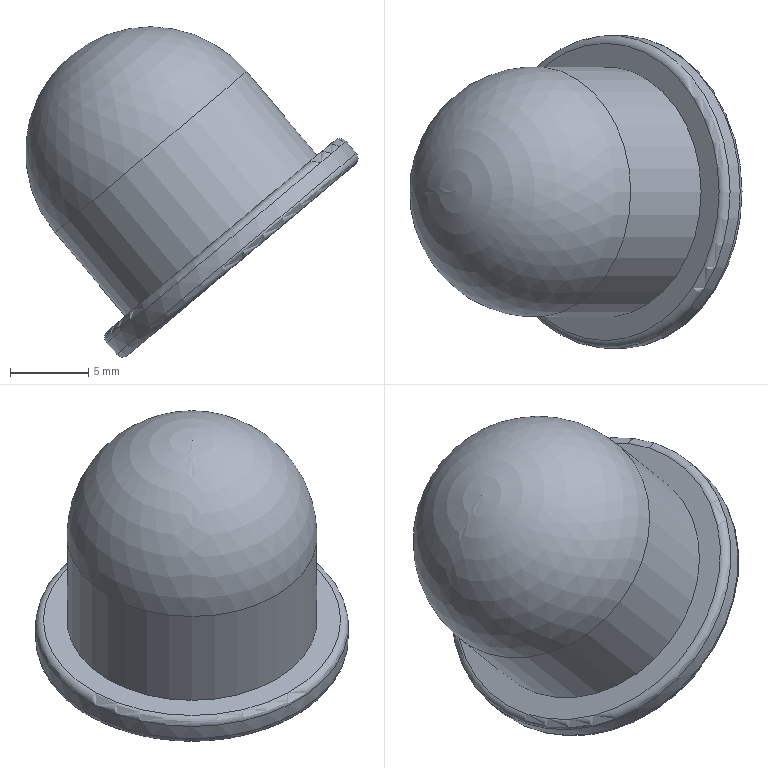Component | NX | PIVOTCUP | 1 solid | 10 faces | box 21.24 x 20 x 21.12 mm | volume 2204 mm3 | cylinder 3 | torus 3 | plane 2 | sphere 2 | commonest cylinder face diameters 16 x1 20 x1 10 x1
STEP:
#1=CARTESIAN_POINT('',(0.,0.,0.));
#2=DIRECTION('',(0.,0.,1.));
#3=DIRECTION('',(1.,0.,0.));
#4=AXIS2_PLACEMENT_3D('',#1,#2,#3);
#5=CARTESIAN_POINT('',(-459.062,-0.,-7.212));
#6=VERTEX_POINT('',#5);
#7=CARTESIAN_POINT('',(-471.318,-0.,-17.497));
#8=VERTEX_POINT('',#7);
#9=CARTESIAN_POINT('',(-465.19,-0.,-12.354));
#10=DIRECTION('',(0.6428,0.,-0.766));
#11=DIRECTION('',(0.766,0.,0.6428));
#12=AXIS2_PLACEMENT_3D('',#9,#10,#11);
#13=CIRCLE('',#12,8.);
#14=CARTESIAN_POINT('',(-470.332,-0.,-6.226));
#15=DIRECTION('',(0.6428,0.,-0.766));
#16=DIRECTION('',(0.766,0.,0.6428));
#17=AXIS2_PLACEMENT_3D('',#14,#15,#16);
#18=CYLINDRICAL_SURFACE('',#17,8.);
#19=CARTESIAN_POINT('',(0.,8.));
#20=DIRECTION('',(1.,0.));
#21=VECTOR('',#20,1.);
#22=LINE('',#19,#21);
#23=(GEOMETRIC_REPRESENTATION_CONTEXT(2)PARAMETRIC_REPRESENTATION_CONTEXT()REPRESENTATION_CONTEXT('',''));
#24=DEFINITIONAL_REPRESENTATION('',(#22),#23);
#25=PCURVE('',#18,#24);
#26=CARTESIAN_POINT('',(-465.19,-0.,-12.354));
#27=DIRECTION('',(-0.6428,0.,0.766));
#28=DIRECTION('',(-0.766,0.,-0.6428));
#29=AXIS2_PLACEMENT_3D('',#26,#27,#28);
#30=SPHERICAL_SURFACE('',#29,8.);
#31=CARTESIAN_POINT('',(3.142,-0.));
#32=CARTESIAN_POINT('',(3.046,0.));
#33=CARTESIAN_POINT('',(2.856,0.));
#34=CARTESIAN_POINT('',(2.57,-0.));
#35=CARTESIAN_POINT('',(2.285,-0.));
#36=CARTESIAN_POINT('',(1.999,-0.));
#37=CARTESIAN_POINT('',(1.714,-0.));
#38=CARTESIAN_POINT('',(1.428,0.));
#39=CARTESIAN_POINT('',(1.142,-0.));
#40=CARTESIAN_POINT('',(0.8568,0.));
#41=CARTESIAN_POINT('',(0.5712,0.));
#42=CARTESIAN_POINT('',(0.2856,-0.));
#43=CARTESIAN_POINT('',(0.,-0.));
#44=CARTESIAN_POINT('',(-0.2856,-0.));
#45=CARTESIAN_POINT('',(-0.5712,0.));
#46=CARTESIAN_POINT('',(-0.8568,0.));
#47=CARTESIAN_POINT('',(-1.142,-0.));
#48=CARTESIAN_POINT('',(-1.428,0.));
#49=CARTESIAN_POINT('',(-1.714,-0.));
#50=CARTESIAN_POINT('',(-1.999,-0.));
#51=CARTESIAN_POINT('',(-2.285,-0.));
#52=CARTESIAN_POINT('',(-2.57,-0.));
#53=CARTESIAN_POINT('',(-2.856,0.));
#54=CARTESIAN_POINT('',(-3.046,0.));
#55=CARTESIAN_POINT('',(-3.142,-0.));
#56=B_SPLINE_CURVE_WITH_KNOTS('',3,(#31,#32,#33,#34,#35,#36,#37,#38,#39,#40,#41,#42,#43,#44,#45,#46,#47,#48,#49,#50,#51,#52,#53,#54,#55),.UNSPECIFIED.,.F.,.F.,(4,1,1,1,1,1,1,1,1,1,1,1,1,1,1,1,1,1,1,1,1,1,4),(0.,0.2856,0.5712,0.8568,1.142,1.428,1.714,1.999,2.285,2.57,2.856,3.142,3.427,3.713,3.998,4.284,4.57,4.855,5.141,5.426,5.712,5.998,6.283),.QUASI_UNIFORM_KNOTS.);
#57=(GEOMETRIC_REPRESENTATION_CONTEXT(2)PARAMETRIC_REPRESENTATION_CONTEXT()REPRESENTATION_CONTEXT('',''));
#58=DEFINITIONAL_REPRESENTATION('',(#56),#57);
#59=PCURVE('',#30,#58);
#60=SURFACE_CURVE('',#13,(#25,#59),.PCURVE_S1.);
#61=EDGE_CURVE('',#6,#8,#60,.T.);
#62=ORIENTED_EDGE('',*,*,#61,.T.);
#63=CARTESIAN_POINT('',(-465.19,-0.,-12.354));
#64=DIRECTION('',(0.6428,0.,-0.766));
#65=DIRECTION('',(0.766,0.,0.6428));
#66=AXIS2_PLACEMENT_3D('',#63,#64,#65);
#67=CIRCLE('',#66,8.);
#68=CARTESIAN_POINT('',(0.,8.));
#69=DIRECTION('',(1.,0.));
#70=VECTOR('',#69,1.);
#71=LINE('',#68,#70);
#72=(GEOMETRIC_REPRESENTATION_CONTEXT(2)PARAMETRIC_REPRESENTATION_CONTEXT()REPRESENTATION_CONTEXT('',''));
#73=DEFINITIONAL_REPRESENTATION('',(#71),#72);
#74=PCURVE('',#18,#73);
#75=CARTESIAN_POINT('',(9.425,-0.));
#76=CARTESIAN_POINT('',(9.33,0.));
#77=CARTESIAN_POINT('',(9.139,0.));
#78=CARTESIAN_POINT('',(8.854,-0.));
#79=CARTESIAN_POINT('',(8.568,-0.));
#80=CARTESIAN_POINT('',(8.282,-0.));
#81=CARTESIAN_POINT('',(7.997,-0.));
#82=CARTESIAN_POINT('',(7.711,0.));
#83=CARTESIAN_POINT('',(7.426,-0.));
#84=CARTESIAN_POINT('',(7.14,0.));
#85=CARTESIAN_POINT('',(6.854,0.));
#86=CARTESIAN_POINT('',(6.569,-0.));
#87=CARTESIAN_POINT('',(6.283,-0.));
#88=CARTESIAN_POINT('',(5.998,-0.));
#89=CARTESIAN_POINT('',(5.712,0.));
#90=CARTESIAN_POINT('',(5.426,0.));
#91=CARTESIAN_POINT('',(5.141,-0.));
#92=CARTESIAN_POINT('',(4.855,0.));
#93=CARTESIAN_POINT('',(4.57,-0.));
#94=CARTESIAN_POINT('',(4.284,-0.));
#95=CARTESIAN_POINT('',(3.998,-0.));
#96=CARTESIAN_POINT('',(3.713,-0.));
#97=CARTESIAN_POINT('',(3.427,0.));
#98=CARTESIAN_POINT('',(3.237,0.));
#99=CARTESIAN_POINT('',(3.142,-0.));
#100=B_SPLINE_CURVE_WITH_KNOTS('',3,(#75,#76,#77,#78,#79,#80,#81,#82,#83,#84,#85,#86,#87,#88,#89,#90,#91,#92,#93,#94,#95,#96,#97,#98,#99),.UNSPECIFIED.,.F.,.F.,(4,1,1,1,1,1,1,1,1,1,1,1,1,1,1,1,1,1,1,1,1,1,4),(0.,0.2856,0.5712,0.8568,1.142,1.428,1.714,1.999,2.285,2.57,2.856,3.142,3.427,3.713,3.998,4.284,4.57,4.855,5.141,5.426,5.712,5.998,6.283),.QUASI_UNIFORM_KNOTS.);
#101=(GEOMETRIC_REPRESENTATION_CONTEXT(2)PARAMETRIC_REPRESENTATION_CONTEXT()REPRESENTATION_CONTEXT('',''));
#102=DEFINITIONAL_REPRESENTATION('',(#100),#101);
#103=PCURVE('',#30,#102);
#104=SURFACE_CURVE('',#67,(#74,#103),.PCURVE_S1.);
#105=EDGE_CURVE('',#8,#6,#104,.T.);
#106=ORIENTED_EDGE('',*,*,#105,.T.);
#107=CARTESIAN_POINT('',(-454.562,-0.,-12.574));
#108=VERTEX_POINT('',#107);
#109=CARTESIAN_POINT('',(-459.062,-0.,-7.212));
#110=CARTESIAN_POINT('',(-454.562,-0.,-12.574));
#111=B_SPLINE_CURVE_WITH_KNOTS('',1,(#109,#110),.UNSPECIFIED.,.F.,.F.,(2,2),(8.,15.),.PIECEWISE_BEZIER_KNOTS.);
#112=CARTESIAN_POINT('',(6.283,0.));
#113=DIRECTION('',(0.,1.));
#114=VECTOR('',#113,1.);
#115=LINE('',#112,#114);
#116=(GEOMETRIC_REPRESENTATION_CONTEXT(2)PARAMETRIC_REPRESENTATION_CONTEXT()REPRESENTATION_CONTEXT('',''));
#117=DEFINITIONAL_REPRESENTATION('',(#115),#116);
#118=PCURVE('',#18,#117);
#119=CARTESIAN_POINT('',(0.,0.));
#120=DIRECTION('',(0.,1.));
#121=VECTOR('',#120,1.);
#122=LINE('',#119,#121);
#123=(GEOMETRIC_REPRESENTATION_CONTEXT(2)PARAMETRIC_REPRESENTATION_CONTEXT()REPRESENTATION_CONTEXT('',''));
#124=DEFINITIONAL_REPRESENTATION('',(#122),#123);
#125=PCURVE('',#18,#124);
#126=SEAM_CURVE('',#111,(#118,#125),.PCURVE_S1.);
#127=EDGE_CURVE('',#6,#108,#126,.T.);
#128=ORIENTED_EDGE('',*,*,#127,.T.);
#129=CARTESIAN_POINT('',(-466.819,-0.,-22.859));
#130=VERTEX_POINT('',#129);
#131=CARTESIAN_POINT('',(-460.69,-0.,-17.717));
#132=DIRECTION('',(0.6428,0.,-0.766));
#133=DIRECTION('',(-0.766,0.,-0.6428));
#134=AXIS2_PLACEMENT_3D('',#131,#132,#133);
#135=CIRCLE('',#134,8.);
#136=CARTESIAN_POINT('',(3.142,15.));
#137=DIRECTION('',(1.,0.));
#138=VECTOR('',#137,1.);
#139=LINE('',#136,#138);
#140=(GEOMETRIC_REPRESENTATION_CONTEXT(2)PARAMETRIC_REPRESENTATION_CONTEXT()REPRESENTATION_CONTEXT('',''));
#141=DEFINITIONAL_REPRESENTATION('',(#139),#140);
#142=PCURVE('',#18,#141);
#143=CARTESIAN_POINT('',(-460.69,-0.,-17.717));
#144=DIRECTION('',(-0.6428,0.,0.766));
#145=DIRECTION('',(-0.766,0.,-0.6428));
#146=AXIS2_PLACEMENT_3D('',#143,#144,#145);
#147=PLANE('',#146);
#148=CARTESIAN_POINT('',(8.,0.));
#149=CARTESIAN_POINT('',(8.,-13.856));
#150=CARTESIAN_POINT('',(-4.,-6.928));
#151=CARTESIAN_POINT('',(-16.,-0.));
#152=CARTESIAN_POINT('',(-4.,6.928));
#153=CARTESIAN_POINT('',(8.,13.856));
#154=CARTESIAN_POINT('',(8.,0.));
#155=(BOUNDED_CURVE()B_SPLINE_CURVE(2,(#148,#149,#150,#151,#152,#153,#154),.UNSPECIFIED.,.T.,.F.)B_SPLINE_CURVE_WITH_KNOTS((1,2,2,2,2,1),(-2.094,0.,2.094,4.189,6.283,8.378),.UNSPECIFIED.)CURVE()GEOMETRIC_REPRESENTATION_ITEM()RATIONAL_B_SPLINE_CURVE((1.,0.5,1.,0.5,1.,0.5,1.))REPRESENTATION_ITEM(''));
#156=(GEOMETRIC_REPRESENTATION_CONTEXT(2)PARAMETRIC_REPRESENTATION_CONTEXT()REPRESENTATION_CONTEXT('',''));
#157=DEFINITIONAL_REPRESENTATION('',(#155),#156);
#158=PCURVE('',#147,#157);
#159=SURFACE_CURVE('',#135,(#142,#158),.PCURVE_S1.);
#160=EDGE_CURVE('',#130,#108,#159,.T.);
#161=ORIENTED_EDGE('',*,*,#160,.F.);
#162=CARTESIAN_POINT('',(-460.69,-0.,-17.717));
#163=DIRECTION('',(0.6428,0.,-0.766));
#164=DIRECTION('',(-0.766,0.,-0.6428));
#165=AXIS2_PLACEMENT_3D('',#162,#163,#164);
#166=CIRCLE('',#165,8.);
#167=CARTESIAN_POINT('',(-3.142,15.));
#168=DIRECTION('',(1.,0.));
#169=VECTOR('',#168,1.);
#170=LINE('',#167,#169);
#171=(GEOMETRIC_REPRESENTATION_CONTEXT(2)PARAMETRIC_REPRESENTATION_CONTEXT()REPRESENTATION_CONTEXT('',''));
#172=DEFINITIONAL_REPRESENTATION('',(#170),#171);
#173=PCURVE('',#18,#172);
#174=CARTESIAN_POINT('',(8.,0.));
#175=CARTESIAN_POINT('',(8.,-13.856));
#176=CARTESIAN_POINT('',(-4.,-6.928));
#177=CARTESIAN_POINT('',(-16.,-0.));
#178=CARTESIAN_POINT('',(-4.,6.928));
#179=CARTESIAN_POINT('',(8.,13.856));
#180=CARTESIAN_POINT('',(8.,0.));
#181=(BOUNDED_CURVE()B_SPLINE_CURVE(2,(#174,#175,#176,#177,#178,#179,#180),.UNSPECIFIED.,.T.,.F.)B_SPLINE_CURVE_WITH_KNOTS((1,2,2,2,2,1),(-2.094,0.,2.094,4.189,6.283,8.378),.UNSPECIFIED.)CURVE()GEOMETRIC_REPRESENTATION_ITEM()RATIONAL_B_SPLINE_CURVE((1.,0.5,1.,0.5,1.,0.5,1.))REPRESENTATION_ITEM(''));
#182=(GEOMETRIC_REPRESENTATION_CONTEXT(2)PARAMETRIC_REPRESENTATION_CONTEXT()REPRESENTATION_CONTEXT('',''));
#183=DEFINITIONAL_REPRESENTATION('',(#181),#182);
#184=PCURVE('',#147,#183);
#185=SURFACE_CURVE('',#166,(#173,#184),.PCURVE_S1.);
#186=EDGE_CURVE('',#108,#130,#185,.T.);
#187=ORIENTED_EDGE('',*,*,#186,.F.);
#188=ORIENTED_EDGE('',*,*,#127,.F.);
#189=EDGE_LOOP('',(#62,#106,#128,#161,#187,#188));
#190=FACE_BOUND('',#189,.T.);
#191=ADVANCED_FACE('',(#190),#18,.T.);
#192=CARTESIAN_POINT('',(-454.809,-0.,-15.392));
#193=VERTEX_POINT('',#192);
#194=CARTESIAN_POINT('',(-459.405,-0.,-19.249));
#195=DIRECTION('',(-0.6428,0.,0.766));
#196=DIRECTION('',(0.766,0.,0.6428));
#197=AXIS2_PLACEMENT_3D('',#194,#195,#196);
#198=CIRCLE('',#197,6.);
#199=CARTESIAN_POINT('',(-459.405,-0.,-19.249));
#200=DIRECTION('',(0.6428,0.,-0.766));
#201=DIRECTION('',(0.766,0.,0.6428));
#202=AXIS2_PLACEMENT_3D('',#199,#200,#201);
#203=PLANE('',#202);
#204=CARTESIAN_POINT('',(6.,0.));
#205=CARTESIAN_POINT('',(6.,-10.392));
#206=CARTESIAN_POINT('',(-3.,-5.196));
#207=CARTESIAN_POINT('',(-12.,-0.));
#208=CARTESIAN_POINT('',(-3.,5.196));
#209=CARTESIAN_POINT('',(6.,10.392));
#210=CARTESIAN_POINT('',(6.,0.));
#211=(BOUNDED_CURVE()B_SPLINE_CURVE(2,(#204,#205,#206,#207,#208,#209,#210),.UNSPECIFIED.,.T.,.F.)B_SPLINE_CURVE_WITH_KNOTS((1,2,2,2,2,1),(-2.094,0.,2.094,4.189,6.283,8.378),.UNSPECIFIED.)CURVE()GEOMETRIC_REPRESENTATION_ITEM()RATIONAL_B_SPLINE_CURVE((1.,0.5,1.,0.5,1.,0.5,1.))REPRESENTATION_ITEM(''));
#212=(GEOMETRIC_REPRESENTATION_CONTEXT(2)PARAMETRIC_REPRESENTATION_CONTEXT()REPRESENTATION_CONTEXT('',''));
#213=DEFINITIONAL_REPRESENTATION('',(#211),#212);
#214=PCURVE('',#203,#213);
#215=CARTESIAN_POINT('',(-460.048,-0.,-18.483));
#216=DIRECTION('',(0.6428,0.,-0.766));
#217=DIRECTION('',(0.766,0.,0.6428));
#218=AXIS2_PLACEMENT_3D('',#215,#216,#217);
#219=TOROIDAL_SURFACE('',#218,6.,1.);
#220=CARTESIAN_POINT('',(6.283,7.854));
#221=DIRECTION('',(-1.,0.));
#222=VECTOR('',#221,1.);
#223=LINE('',#220,#222);
#224=(GEOMETRIC_REPRESENTATION_CONTEXT(2)PARAMETRIC_REPRESENTATION_CONTEXT()REPRESENTATION_CONTEXT('',''));
#225=DEFINITIONAL_REPRESENTATION('',(#223),#224);
#226=PCURVE('',#219,#225);
#227=SURFACE_CURVE('',#198,(#214,#226),.PCURVE_S1.);
#228=EDGE_CURVE('',#193,#193,#227,.T.);
#229=ORIENTED_EDGE('',*,*,#228,.T.);
#230=EDGE_LOOP('',(#229));
#231=FACE_BOUND('',#230,.T.);
#232=CARTESIAN_POINT('',(-452.127,-0.,-13.142));
#233=VERTEX_POINT('',#232);
#234=CARTESIAN_POINT('',(-459.405,-0.,-19.249));
#235=DIRECTION('',(0.6428,0.,-0.766));
#236=DIRECTION('',(0.766,0.,0.6428));
#237=AXIS2_PLACEMENT_3D('',#234,#235,#236);
#238=CIRCLE('',#237,9.5);
#239=CARTESIAN_POINT('',(0.,0.));
#240=DIRECTION('',(1.,0.));
#241=AXIS2_PLACEMENT_2D('',#239,#240);
#242=CIRCLE('',#241,9.5);
#243=(GEOMETRIC_REPRESENTATION_CONTEXT(2)PARAMETRIC_REPRESENTATION_CONTEXT()REPRESENTATION_CONTEXT('',''));
#244=DEFINITIONAL_REPRESENTATION('',(#242),#243);
#245=PCURVE('',#203,#244);
#246=CARTESIAN_POINT('',(-459.726,-0.,-18.866));
#247=DIRECTION('',(0.6428,0.,-0.766));
#248=DIRECTION('',(0.766,0.,0.6428));
#249=AXIS2_PLACEMENT_3D('',#246,#247,#248);
#250=TOROIDAL_SURFACE('',#249,9.5,0.5);
#251=CARTESIAN_POINT('',(0.,7.854));
#252=DIRECTION('',(1.,0.));
#253=VECTOR('',#252,1.);
#254=LINE('',#251,#253);
#255=(GEOMETRIC_REPRESENTATION_CONTEXT(2)PARAMETRIC_REPRESENTATION_CONTEXT()REPRESENTATION_CONTEXT('',''));
#256=DEFINITIONAL_REPRESENTATION('',(#254),#255);
#257=PCURVE('',#250,#256);
#258=SURFACE_CURVE('',#238,(#245,#257),.PCURVE_S1.);
#259=EDGE_CURVE('',#233,#233,#258,.T.);
#260=ORIENTED_EDGE('',*,*,#259,.T.);
#261=EDGE_LOOP('',(#260));
#262=FACE_BOUND('',#261,.T.);
#263=ADVANCED_FACE('',(#231,#262),#203,.T.);
#264=CARTESIAN_POINT('',(-467.968,-0.,-23.823));
#265=VERTEX_POINT('',#264);
#266=CARTESIAN_POINT('',(-460.69,-0.,-17.717));
#267=DIRECTION('',(-0.6428,0.,0.766));
#268=DIRECTION('',(-0.766,0.,-0.6428));
#269=AXIS2_PLACEMENT_3D('',#266,#267,#268);
#270=CIRCLE('',#269,9.5);
#271=CARTESIAN_POINT('',(0.,0.));
#272=DIRECTION('',(1.,0.));
#273=AXIS2_PLACEMENT_2D('',#271,#272);
#274=CIRCLE('',#273,9.5);
#275=(GEOMETRIC_REPRESENTATION_CONTEXT(2)PARAMETRIC_REPRESENTATION_CONTEXT()REPRESENTATION_CONTEXT('',''));
#276=DEFINITIONAL_REPRESENTATION('',(#274),#275);
#277=PCURVE('',#147,#276);
#278=CARTESIAN_POINT('',(-460.369,-0.,-18.1));
#279=DIRECTION('',(-0.6428,0.,0.766));
#280=DIRECTION('',(-0.766,0.,-0.6428));
#281=AXIS2_PLACEMENT_3D('',#278,#279,#280);
#282=TOROIDAL_SURFACE('',#281,9.5,0.5);
#283=CARTESIAN_POINT('',(0.,7.854));
#284=DIRECTION('',(1.,0.));
#285=VECTOR('',#284,1.);
#286=LINE('',#283,#285);
#287=(GEOMETRIC_REPRESENTATION_CONTEXT(2)PARAMETRIC_REPRESENTATION_CONTEXT()REPRESENTATION_CONTEXT('',''));
#288=DEFINITIONAL_REPRESENTATION('',(#286),#287);
#289=PCURVE('',#282,#288);
#290=SURFACE_CURVE('',#270,(#277,#289),.PCURVE_S1.);
#291=EDGE_CURVE('',#265,#265,#290,.T.);
#292=ORIENTED_EDGE('',*,*,#291,.T.);
#293=EDGE_LOOP('',(#292));
#294=FACE_BOUND('',#293,.T.);
#295=ORIENTED_EDGE('',*,*,#160,.T.);
#296=ORIENTED_EDGE('',*,*,#186,.T.);
#297=EDGE_LOOP('',(#295,#296));
#298=FACE_BOUND('',#297,.T.);
#299=ADVANCED_FACE('',(#294,#298),#147,.T.);
#300=CARTESIAN_POINT('',(-452.066,-0.,-12.438));
#301=VERTEX_POINT('',#300);
#302=CARTESIAN_POINT('',(-459.726,-0.,-18.866));
#303=DIRECTION('',(-0.6428,0.,0.766));
#304=DIRECTION('',(0.766,0.,0.6428));
#305=AXIS2_PLACEMENT_3D('',#302,#303,#304);
#306=CIRCLE('',#305,10.);
#307=CARTESIAN_POINT('',(-460.69,-0.,-17.717));
#308=DIRECTION('',(0.6428,0.,-0.766));
#309=DIRECTION('',(0.766,0.,0.6428));
#310=AXIS2_PLACEMENT_3D('',#307,#308,#309);
#311=CYLINDRICAL_SURFACE('',#310,10.);
#312=CARTESIAN_POINT('',(6.283,1.5));
#313=DIRECTION('',(-1.,0.));
#314=VECTOR('',#313,1.);
#315=LINE('',#312,#314);
#316=(GEOMETRIC_REPRESENTATION_CONTEXT(2)PARAMETRIC_REPRESENTATION_CONTEXT()REPRESENTATION_CONTEXT('',''));
#317=DEFINITIONAL_REPRESENTATION('',(#315),#316);
#318=PCURVE('',#311,#317);
#319=CARTESIAN_POINT('',(6.283,6.283));
#320=DIRECTION('',(-1.,0.));
#321=VECTOR('',#320,1.);
#322=LINE('',#319,#321);
#323=(GEOMETRIC_REPRESENTATION_CONTEXT(2)PARAMETRIC_REPRESENTATION_CONTEXT()REPRESENTATION_CONTEXT('',''));
#324=DEFINITIONAL_REPRESENTATION('',(#322),#323);
#325=PCURVE('',#250,#324);
#326=SURFACE_CURVE('',#306,(#318,#325),.PCURVE_S1.);
#327=EDGE_CURVE('',#301,#301,#326,.T.);
#328=ORIENTED_EDGE('',*,*,#327,.T.);
#329=CARTESIAN_POINT('',(-452.709,-0.,-11.672));
#330=VERTEX_POINT('',#329);
#331=CARTESIAN_POINT('',(-452.709,-0.,-11.672));
#332=CARTESIAN_POINT('',(-452.066,-0.,-12.438));
#333=B_SPLINE_CURVE_WITH_KNOTS('',1,(#331,#332),.UNSPECIFIED.,.F.,.F.,(2,2),(0.5,1.5),.PIECEWISE_BEZIER_KNOTS.);
#334=CARTESIAN_POINT('',(0.,0.));
#335=DIRECTION('',(0.,1.));
#336=VECTOR('',#335,1.);
#337=LINE('',#334,#336);
#338=(GEOMETRIC_REPRESENTATION_CONTEXT(2)PARAMETRIC_REPRESENTATION_CONTEXT()REPRESENTATION_CONTEXT('',''));
#339=DEFINITIONAL_REPRESENTATION('',(#337),#338);
#340=PCURVE('',#311,#339);
#341=CARTESIAN_POINT('',(6.283,0.));
#342=DIRECTION('',(0.,1.));
#343=VECTOR('',#342,1.);
#344=LINE('',#341,#343);
#345=(GEOMETRIC_REPRESENTATION_CONTEXT(2)PARAMETRIC_REPRESENTATION_CONTEXT()REPRESENTATION_CONTEXT('',''));
#346=DEFINITIONAL_REPRESENTATION('',(#344),#345);
#347=PCURVE('',#311,#346);
#348=SEAM_CURVE('',#333,(#340,#347),.PCURVE_S1.);
#349=EDGE_CURVE('',#330,#301,#348,.T.);
#350=ORIENTED_EDGE('',*,*,#349,.F.);
#351=CARTESIAN_POINT('',(-468.029,-0.,-24.527));
#352=VERTEX_POINT('',#351);
#353=CARTESIAN_POINT('',(-460.369,-0.,-18.1));
#354=DIRECTION('',(0.6428,0.,-0.766));
#355=DIRECTION('',(-0.766,0.,-0.6428));
#356=AXIS2_PLACEMENT_3D('',#353,#354,#355);
#357=CIRCLE('',#356,10.);
#358=CARTESIAN_POINT('',(-3.142,0.5));
#359=DIRECTION('',(1.,0.));
#360=VECTOR('',#359,1.);
#361=LINE('',#358,#360);
#362=(GEOMETRIC_REPRESENTATION_CONTEXT(2)PARAMETRIC_REPRESENTATION_CONTEXT()REPRESENTATION_CONTEXT('',''));
#363=DEFINITIONAL_REPRESENTATION('',(#361),#362);
#364=PCURVE('',#311,#363);
#365=CARTESIAN_POINT('',(6.283,6.283));
#366=DIRECTION('',(-1.,0.));
#367=VECTOR('',#366,1.);
#368=LINE('',#365,#367);
#369=(GEOMETRIC_REPRESENTATION_CONTEXT(2)PARAMETRIC_REPRESENTATION_CONTEXT()REPRESENTATION_CONTEXT('',''));
#370=DEFINITIONAL_REPRESENTATION('',(#368),#369);
#371=PCURVE('',#282,#370);
#372=SURFACE_CURVE('',#357,(#364,#371),.PCURVE_S1.);
#373=EDGE_CURVE('',#330,#352,#372,.T.);
#374=ORIENTED_EDGE('',*,*,#373,.T.);
#375=CARTESIAN_POINT('',(-460.369,-0.,-18.1));
#376=DIRECTION('',(0.6428,0.,-0.766));
#377=DIRECTION('',(-0.766,0.,-0.6428));
#378=AXIS2_PLACEMENT_3D('',#375,#376,#377);
#379=CIRCLE('',#378,10.);
#380=CARTESIAN_POINT('',(3.142,0.5));
#381=DIRECTION('',(1.,0.));
#382=VECTOR('',#381,1.);
#383=LINE('',#380,#382);
#384=(GEOMETRIC_REPRESENTATION_CONTEXT(2)PARAMETRIC_REPRESENTATION_CONTEXT()REPRESENTATION_CONTEXT('',''));
#385=DEFINITIONAL_REPRESENTATION('',(#383),#384);
#386=PCURVE('',#311,#385);
#387=CARTESIAN_POINT('',(6.283,6.283));
#388=DIRECTION('',(-1.,0.));
#389=VECTOR('',#388,1.);
#390=LINE('',#387,#389);
#391=(GEOMETRIC_REPRESENTATION_CONTEXT(2)PARAMETRIC_REPRESENTATION_CONTEXT()REPRESENTATION_CONTEXT('',''));
#392=DEFINITIONAL_REPRESENTATION('',(#390),#391);
#393=PCURVE('',#282,#392);
#394=SURFACE_CURVE('',#379,(#386,#393),.PCURVE_S1.);
#395=EDGE_CURVE('',#352,#330,#394,.T.);
#396=ORIENTED_EDGE('',*,*,#395,.T.);
#397=ORIENTED_EDGE('',*,*,#349,.T.);
#398=EDGE_LOOP('',(#328,#350,#374,#396,#397));
#399=FACE_BOUND('',#398,.T.);
#400=ADVANCED_FACE('',(#399),#311,.T.);
#401=ORIENTED_EDGE('',*,*,#259,.F.);
#402=CARTESIAN_POINT('',(-452.066,-0.,-12.438));
#403=CARTESIAN_POINT('',(-451.98,-0.,-12.54));
#404=CARTESIAN_POINT('',(-451.929,-0.,-12.667));
#405=CARTESIAN_POINT('',(-451.919,-0.,-12.805));
#406=CARTESIAN_POINT('',(-451.953,-0.,-12.94));
#407=CARTESIAN_POINT('',(-452.025,-0.,-13.056));
#408=CARTESIAN_POINT('',(-452.127,-0.,-13.142));
#409=(BOUNDED_CURVE()B_SPLINE_CURVE(6,(#402,#403,#404,#405,#406,#407,#408),.UNSPECIFIED.,.F.,.F.)B_SPLINE_CURVE_WITH_KNOTS((7,7),(0.,1.571),.PIECEWISE_BEZIER_KNOTS.)CURVE()GEOMETRIC_REPRESENTATION_ITEM()RATIONAL_B_SPLINE_CURVE((1.031,1.01,0.9979,0.994,0.9979,1.01,1.031))REPRESENTATION_ITEM(''));
#410=CARTESIAN_POINT('',(0.,6.283));
#411=DIRECTION('',(0.,1.));
#412=VECTOR('',#411,1.);
#413=LINE('',#410,#412);
#414=(GEOMETRIC_REPRESENTATION_CONTEXT(2)PARAMETRIC_REPRESENTATION_CONTEXT()REPRESENTATION_CONTEXT('',''));
#415=DEFINITIONAL_REPRESENTATION('',(#413),#414);
#416=PCURVE('',#250,#415);
#417=CARTESIAN_POINT('',(6.283,6.283));
#418=DIRECTION('',(0.,1.));
#419=VECTOR('',#418,1.);
#420=LINE('',#417,#419);
#421=(GEOMETRIC_REPRESENTATION_CONTEXT(2)PARAMETRIC_REPRESENTATION_CONTEXT()REPRESENTATION_CONTEXT('',''));
#422=DEFINITIONAL_REPRESENTATION('',(#420),#421);
#423=PCURVE('',#250,#422);
#424=SEAM_CURVE('',#409,(#416,#423),.PCURVE_S1.);
#425=EDGE_CURVE('',#301,#233,#424,.T.);
#426=ORIENTED_EDGE('',*,*,#425,.F.);
#427=ORIENTED_EDGE('',*,*,#327,.F.);
#428=ORIENTED_EDGE('',*,*,#425,.T.);
#429=EDGE_LOOP('',(#401,#426,#427,#428));
#430=FACE_BOUND('',#429,.T.);
#431=ADVANCED_FACE('',(#430),#250,.T.);
#432=ORIENTED_EDGE('',*,*,#291,.F.);
#433=CARTESIAN_POINT('',(-468.029,-0.,-24.527));
#434=CARTESIAN_POINT('',(-468.115,-0.,-24.425));
#435=CARTESIAN_POINT('',(-468.166,-0.,-24.298));
#436=CARTESIAN_POINT('',(-468.176,-0.,-24.16));
#437=CARTESIAN_POINT('',(-468.143,-0.,-24.025));
#438=CARTESIAN_POINT('',(-468.07,-0.,-23.909));
#439=CARTESIAN_POINT('',(-467.968,-0.,-23.823));
#440=(BOUNDED_CURVE()B_SPLINE_CURVE(6,(#433,#434,#435,#436,#437,#438,#439),.UNSPECIFIED.,.F.,.F.)B_SPLINE_CURVE_WITH_KNOTS((7,7),(0.,1.571),.PIECEWISE_BEZIER_KNOTS.)CURVE()GEOMETRIC_REPRESENTATION_ITEM()RATIONAL_B_SPLINE_CURVE((1.031,1.01,0.9979,0.994,0.9979,1.01,1.031))REPRESENTATION_ITEM(''));
#441=CARTESIAN_POINT('',(0.,6.283));
#442=DIRECTION('',(0.,1.));
#443=VECTOR('',#442,1.);
#444=LINE('',#441,#443);
#445=(GEOMETRIC_REPRESENTATION_CONTEXT(2)PARAMETRIC_REPRESENTATION_CONTEXT()REPRESENTATION_CONTEXT('',''));
#446=DEFINITIONAL_REPRESENTATION('',(#444),#445);
#447=PCURVE('',#282,#446);
#448=CARTESIAN_POINT('',(6.283,6.283));
#449=DIRECTION('',(0.,1.));
#450=VECTOR('',#449,1.);
#451=LINE('',#448,#450);
#452=(GEOMETRIC_REPRESENTATION_CONTEXT(2)PARAMETRIC_REPRESENTATION_CONTEXT()REPRESENTATION_CONTEXT('',''));
#453=DEFINITIONAL_REPRESENTATION('',(#451),#452);
#454=PCURVE('',#282,#453);
#455=SEAM_CURVE('',#440,(#447,#454),.PCURVE_S1.);
#456=EDGE_CURVE('',#352,#265,#455,.T.);
#457=ORIENTED_EDGE('',*,*,#456,.F.);
#458=ORIENTED_EDGE('',*,*,#373,.F.);
#459=ORIENTED_EDGE('',*,*,#395,.F.);
#460=ORIENTED_EDGE('',*,*,#456,.T.);
#461=EDGE_LOOP('',(#432,#457,#458,#459,#460));
#462=FACE_BOUND('',#461,.T.);
#463=ADVANCED_FACE('',(#462),#282,.T.);
#464=ORIENTED_EDGE('',*,*,#105,.F.);
#465=CARTESIAN_POINT('',(-470.332,-0.,-6.226));
#466=VERTEX_POINT('',#465);
#467=CARTESIAN_POINT('',(-471.318,-0.,-17.497));
#468=CARTESIAN_POINT('',(-472.472,-0.,-16.121));
#469=CARTESIAN_POINT('',(-473.266,-0.,-14.444));
#470=CARTESIAN_POINT('',(-473.605,-0.,-12.578));
#471=CARTESIAN_POINT('',(-473.438,-0.,-10.673));
#472=CARTESIAN_POINT('',(-472.78,-0.,-8.894));
#473=CARTESIAN_POINT('',(-471.707,-0.,-7.38));
#474=CARTESIAN_POINT('',(-470.332,-0.,-6.226));
#475=B_SPLINE_CURVE_WITH_KNOTS('',7,(#467,#468,#469,#470,#471,#472,#473,#474),.UNSPECIFIED.,.F.,.F.,(8,8),(-0.,1.571),.PIECEWISE_BEZIER_KNOTS.);
#476=CARTESIAN_POINT('',(6.283,0.));
#477=DIRECTION('',(0.,1.));
#478=VECTOR('',#477,1.);
#479=LINE('',#476,#478);
#480=(GEOMETRIC_REPRESENTATION_CONTEXT(2)PARAMETRIC_REPRESENTATION_CONTEXT()REPRESENTATION_CONTEXT('',''));
#481=DEFINITIONAL_REPRESENTATION('',(#479),#480);
#482=PCURVE('',#30,#481);
#483=CARTESIAN_POINT('',(0.,0.));
#484=DIRECTION('',(0.,1.));
#485=VECTOR('',#484,1.);
#486=LINE('',#483,#485);
#487=(GEOMETRIC_REPRESENTATION_CONTEXT(2)PARAMETRIC_REPRESENTATION_CONTEXT()REPRESENTATION_CONTEXT('',''));
#488=DEFINITIONAL_REPRESENTATION('',(#486),#487);
#489=PCURVE('',#30,#488);
#490=SEAM_CURVE('',#475,(#482,#489),.PCURVE_S1.);
#491=EDGE_CURVE('',#8,#466,#490,.T.);
#492=ORIENTED_EDGE('',*,*,#491,.T.);
#493=ORIENTED_EDGE('',*,*,#491,.F.);
#494=ORIENTED_EDGE('',*,*,#61,.F.);
#495=EDGE_LOOP('',(#464,#492,#493,#494));
#496=FACE_BOUND('',#495,.T.);
#497=ADVANCED_FACE('',(#496),#30,.T.);
#498=CARTESIAN_POINT('',(-463.878,-0.,-21.697));
#499=VERTEX_POINT('',#498);
#500=CARTESIAN_POINT('',(-456.217,-0.,-15.269));
#501=VERTEX_POINT('',#500);
#502=CARTESIAN_POINT('',(-460.048,-0.,-18.483));
#503=DIRECTION('',(0.6428,0.,-0.766));
#504=DIRECTION('',(0.766,0.,0.6428));
#505=AXIS2_PLACEMENT_3D('',#502,#503,#504);
#506=CIRCLE('',#505,5.);
#507=CARTESIAN_POINT('',(-459.405,-0.,-19.249));
#508=DIRECTION('',(-0.6428,0.,0.766));
#509=DIRECTION('',(-0.766,0.,-0.6428));
#510=AXIS2_PLACEMENT_3D('',#507,#508,#509);
#511=CYLINDRICAL_SURFACE('',#510,5.);
#512=CARTESIAN_POINT('',(9.425,1.));
#513=DIRECTION('',(-1.,0.));
#514=VECTOR('',#513,1.);
#515=LINE('',#512,#514);
#516=(GEOMETRIC_REPRESENTATION_CONTEXT(2)PARAMETRIC_REPRESENTATION_CONTEXT()REPRESENTATION_CONTEXT('',''));
#517=DEFINITIONAL_REPRESENTATION('',(#515),#516);
#518=PCURVE('',#511,#517);
#519=CARTESIAN_POINT('',(0.,9.425));
#520=DIRECTION('',(1.,0.));
#521=VECTOR('',#520,1.);
#522=LINE('',#519,#521);
#523=(GEOMETRIC_REPRESENTATION_CONTEXT(2)PARAMETRIC_REPRESENTATION_CONTEXT()REPRESENTATION_CONTEXT('',''));
#524=DEFINITIONAL_REPRESENTATION('',(#522),#523);
#525=PCURVE('',#219,#524);
#526=SURFACE_CURVE('',#506,(#518,#525),.PCURVE_S1.);
#527=EDGE_CURVE('',#499,#501,#526,.T.);
#528=ORIENTED_EDGE('',*,*,#527,.F.);
#529=CARTESIAN_POINT('',(-468.377,-0.,-16.334));
#530=VERTEX_POINT('',#529);
#531=CARTESIAN_POINT('',(-463.878,-0.,-21.697));
#532=CARTESIAN_POINT('',(-468.377,-0.,-16.334));
#533=B_SPLINE_CURVE_WITH_KNOTS('',1,(#531,#532),.UNSPECIFIED.,.F.,.F.,(2,2),(1.,8.),.PIECEWISE_BEZIER_KNOTS.);
#534=CARTESIAN_POINT('',(6.283,0.));
#535=DIRECTION('',(0.,1.));
#536=VECTOR('',#535,1.);
#537=LINE('',#534,#536);
#538=(GEOMETRIC_REPRESENTATION_CONTEXT(2)PARAMETRIC_REPRESENTATION_CONTEXT()REPRESENTATION_CONTEXT('',''));
#539=DEFINITIONAL_REPRESENTATION('',(#537),#538);
#540=PCURVE('',#511,#539);
#541=CARTESIAN_POINT('',(0.,0.));
#542=DIRECTION('',(0.,1.));
#543=VECTOR('',#542,1.);
#544=LINE('',#541,#543);
#545=(GEOMETRIC_REPRESENTATION_CONTEXT(2)PARAMETRIC_REPRESENTATION_CONTEXT()REPRESENTATION_CONTEXT('',''));
#546=DEFINITIONAL_REPRESENTATION('',(#544),#545);
#547=PCURVE('',#511,#546);
#548=SEAM_CURVE('',#533,(#540,#547),.PCURVE_S1.);
#549=EDGE_CURVE('',#499,#530,#548,.T.);
#550=ORIENTED_EDGE('',*,*,#549,.T.);
#551=CARTESIAN_POINT('',(-464.547,-0.,-13.12));
#552=DIRECTION('',(-0.6428,0.,0.766));
#553=DIRECTION('',(-0.766,0.,-0.6428));
#554=AXIS2_PLACEMENT_3D('',#551,#552,#553);
#555=CIRCLE('',#554,5.);
#556=CARTESIAN_POINT('',(0.,8.));
#557=DIRECTION('',(1.,0.));
#558=VECTOR('',#557,1.);
#559=LINE('',#556,#558);
#560=(GEOMETRIC_REPRESENTATION_CONTEXT(2)PARAMETRIC_REPRESENTATION_CONTEXT()REPRESENTATION_CONTEXT('',''));
#561=DEFINITIONAL_REPRESENTATION('',(#559),#560);
#562=PCURVE('',#511,#561);
#563=CARTESIAN_POINT('',(-464.547,-0.,-13.12));
#564=DIRECTION('',(-0.6428,0.,0.766));
#565=DIRECTION('',(-0.766,0.,-0.6428));
#566=AXIS2_PLACEMENT_3D('',#563,#564,#565);
#567=SPHERICAL_SURFACE('',#566,5.);
#568=CARTESIAN_POINT('',(0.,0.));
#569=DIRECTION('',(1.,0.));
#570=VECTOR('',#569,1.);
#571=LINE('',#568,#570);
#572=(GEOMETRIC_REPRESENTATION_CONTEXT(2)PARAMETRIC_REPRESENTATION_CONTEXT()REPRESENTATION_CONTEXT('',''));
#573=DEFINITIONAL_REPRESENTATION('',(#571),#572);
#574=PCURVE('',#567,#573);
#575=SURFACE_CURVE('',#555,(#562,#574),.PCURVE_S1.);
#576=EDGE_CURVE('',#530,#530,#575,.T.);
#577=ORIENTED_EDGE('',*,*,#576,.F.);
#578=ORIENTED_EDGE('',*,*,#549,.F.);
#579=CARTESIAN_POINT('',(-460.048,-0.,-18.483));
#580=DIRECTION('',(0.6428,0.,-0.766));
#581=DIRECTION('',(0.766,0.,0.6428));
#582=AXIS2_PLACEMENT_3D('',#579,#580,#581);
#583=CIRCLE('',#582,5.);
#584=CARTESIAN_POINT('',(3.142,1.));
#585=DIRECTION('',(-1.,0.));
#586=VECTOR('',#585,1.);
#587=LINE('',#584,#586);
#588=(GEOMETRIC_REPRESENTATION_CONTEXT(2)PARAMETRIC_REPRESENTATION_CONTEXT()REPRESENTATION_CONTEXT('',''));
#589=DEFINITIONAL_REPRESENTATION('',(#587),#588);
#590=PCURVE('',#511,#589);
#591=CARTESIAN_POINT('',(0.,9.425));
#592=DIRECTION('',(1.,0.));
#593=VECTOR('',#592,1.);
#594=LINE('',#591,#593);
#595=(GEOMETRIC_REPRESENTATION_CONTEXT(2)PARAMETRIC_REPRESENTATION_CONTEXT()REPRESENTATION_CONTEXT('',''));
#596=DEFINITIONAL_REPRESENTATION('',(#594),#595);
#597=PCURVE('',#219,#596);
#598=SURFACE_CURVE('',#583,(#590,#597),.PCURVE_S1.);
#599=EDGE_CURVE('',#501,#499,#598,.T.);
#600=ORIENTED_EDGE('',*,*,#599,.F.);
#601=EDGE_LOOP('',(#528,#550,#577,#578,#600));
#602=FACE_BOUND('',#601,.F.);
#603=ADVANCED_FACE('',(#602),#511,.F.);
#604=ORIENTED_EDGE('',*,*,#599,.F.);
#605=CARTESIAN_POINT('',(-454.809,-0.,-15.392));
#606=CARTESIAN_POINT('',(-455.013,-0.,-15.564));
#607=CARTESIAN_POINT('',(-455.267,-0.,-15.666));
#608=CARTESIAN_POINT('',(-455.544,-0.,-15.685));
#609=CARTESIAN_POINT('',(-455.813,-0.,-15.618));
#610=CARTESIAN_POINT('',(-456.046,-0.,-15.473));
#611=CARTESIAN_POINT('',(-456.217,-0.,-15.269));
#612=(BOUNDED_CURVE()B_SPLINE_CURVE(6,(#605,#606,#607,#608,#609,#610,#611),.UNSPECIFIED.,.F.,.F.)B_SPLINE_CURVE_WITH_KNOTS((7,7),(1.571,3.142),.PIECEWISE_BEZIER_KNOTS.)CURVE()GEOMETRIC_REPRESENTATION_ITEM()RATIONAL_B_SPLINE_CURVE((1.031,1.01,0.9979,0.994,0.9979,1.01,1.031))REPRESENTATION_ITEM(''));
#613=CARTESIAN_POINT('',(0.,6.283));
#614=DIRECTION('',(0.,1.));
#615=VECTOR('',#614,1.);
#616=LINE('',#613,#615);
#617=(GEOMETRIC_REPRESENTATION_CONTEXT(2)PARAMETRIC_REPRESENTATION_CONTEXT()REPRESENTATION_CONTEXT('',''));
#618=DEFINITIONAL_REPRESENTATION('',(#616),#617);
#619=PCURVE('',#219,#618);
#620=CARTESIAN_POINT('',(6.283,6.283));
#621=DIRECTION('',(0.,1.));
#622=VECTOR('',#621,1.);
#623=LINE('',#620,#622);
#624=(GEOMETRIC_REPRESENTATION_CONTEXT(2)PARAMETRIC_REPRESENTATION_CONTEXT()REPRESENTATION_CONTEXT('',''));
#625=DEFINITIONAL_REPRESENTATION('',(#623),#624);
#626=PCURVE('',#219,#625);
#627=SEAM_CURVE('',#612,(#619,#626),.PCURVE_S1.);
#628=EDGE_CURVE('',#193,#501,#627,.T.);
#629=ORIENTED_EDGE('',*,*,#628,.F.);
#630=ORIENTED_EDGE('',*,*,#228,.F.);
#631=ORIENTED_EDGE('',*,*,#628,.T.);
#632=ORIENTED_EDGE('',*,*,#527,.F.);
#633=EDGE_LOOP('',(#604,#629,#630,#631,#632));
#634=FACE_BOUND('',#633,.T.);
#635=ADVANCED_FACE('',(#634),#219,.T.);
#636=ORIENTED_EDGE('',*,*,#576,.T.);
#637=CARTESIAN_POINT('',(-467.761,-0.,-9.29));
#638=VERTEX_POINT('',#637);
#639=CARTESIAN_POINT('',(-468.377,-0.,-16.334));
#640=CARTESIAN_POINT('',(-469.219,-0.,-15.331));
#641=CARTESIAN_POINT('',(-469.745,-0.,-14.065));
#642=CARTESIAN_POINT('',(-469.853,-0.,-12.656));
#643=CARTESIAN_POINT('',(-469.502,-0.,-11.288));
#644=CARTESIAN_POINT('',(-468.764,-0.,-10.131));
#645=CARTESIAN_POINT('',(-467.761,-0.,-9.29));
#646=B_SPLINE_CURVE_WITH_KNOTS('',6,(#639,#640,#641,#642,#643,#644,#645),.UNSPECIFIED.,.F.,.F.,(7,7),(0.,1.571),.PIECEWISE_BEZIER_KNOTS.);
#647=CARTESIAN_POINT('',(6.283,0.));
#648=DIRECTION('',(0.,1.));
#649=VECTOR('',#648,1.);
#650=LINE('',#647,#649);
#651=(GEOMETRIC_REPRESENTATION_CONTEXT(2)PARAMETRIC_REPRESENTATION_CONTEXT()REPRESENTATION_CONTEXT('',''));
#652=DEFINITIONAL_REPRESENTATION('',(#650),#651);
#653=PCURVE('',#567,#652);
#654=CARTESIAN_POINT('',(0.,0.));
#655=DIRECTION('',(0.,1.));
#656=VECTOR('',#655,1.);
#657=LINE('',#654,#656);
#658=(GEOMETRIC_REPRESENTATION_CONTEXT(2)PARAMETRIC_REPRESENTATION_CONTEXT()REPRESENTATION_CONTEXT('',''));
#659=DEFINITIONAL_REPRESENTATION('',(#657),#658);
#660=PCURVE('',#567,#659);
#661=SEAM_CURVE('',#646,(#653,#660),.PCURVE_S1.);
#662=EDGE_CURVE('',#530,#638,#661,.T.);
#663=ORIENTED_EDGE('',*,*,#662,.T.);
#664=ORIENTED_EDGE('',*,*,#662,.F.);
#665=EDGE_LOOP('',(#636,#663,#664));
#666=FACE_BOUND('',#665,.F.);
#667=ADVANCED_FACE('',(#666),#567,.F.);
#668=CLOSED_SHELL('',(#191,#263,#299,#400,#431,#463,#497,#603,#635,#667));
#669=MANIFOLD_SOLID_BREP('',#668);
#670=(LENGTH_UNIT()NAMED_UNIT(*)SI_UNIT(.MILLI.,.METRE.));
#671=UNCERTAINTY_MEASURE_WITH_UNIT(LENGTH_MEASURE(0.00001),#670,'','');
#672=(NAMED_UNIT(*)PLANE_ANGLE_UNIT()SI_UNIT($,.RADIAN.));
#673=(NAMED_UNIT(*)SI_UNIT($,.STERADIAN.)SOLID_ANGLE_UNIT());
#674=(GEOMETRIC_REPRESENTATION_CONTEXT(3)GLOBAL_UNCERTAINTY_ASSIGNED_CONTEXT((#671))GLOBAL_UNIT_ASSIGNED_CONTEXT((#670,#672,#673))REPRESENTATION_CONTEXT('',''));
#675=ADVANCED_BREP_SHAPE_REPRESENTATION('',(#4,#669),#674);